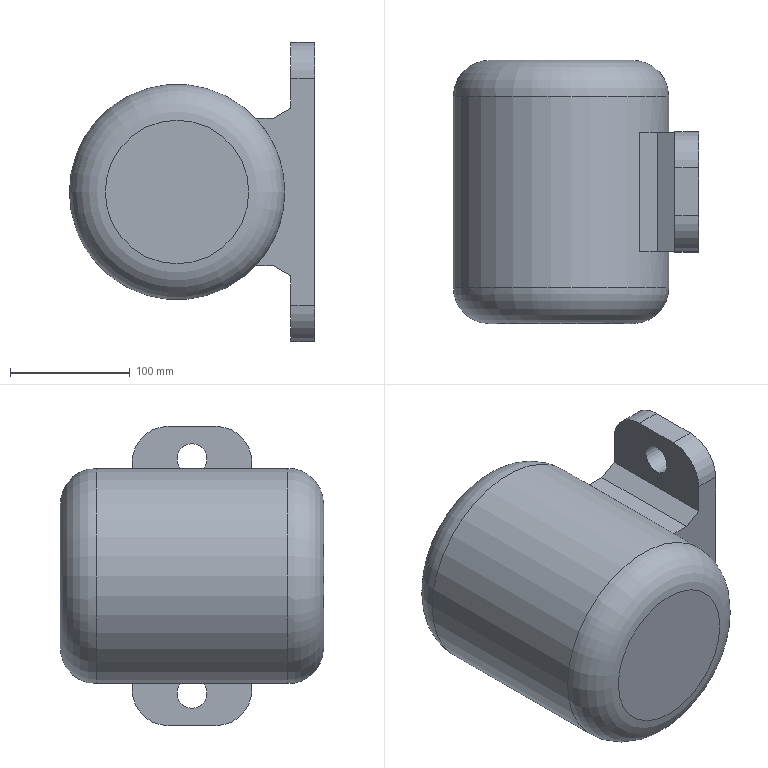Component | NX | MOTOR_MOUNT | 1 solid | 28 faces | volume 3268846 mm3 | plane 15 | cylinder 9 | torus 4 | commonest cylinder face diameters 60 x4 25 x2 180 x1 140 x1 22 x1